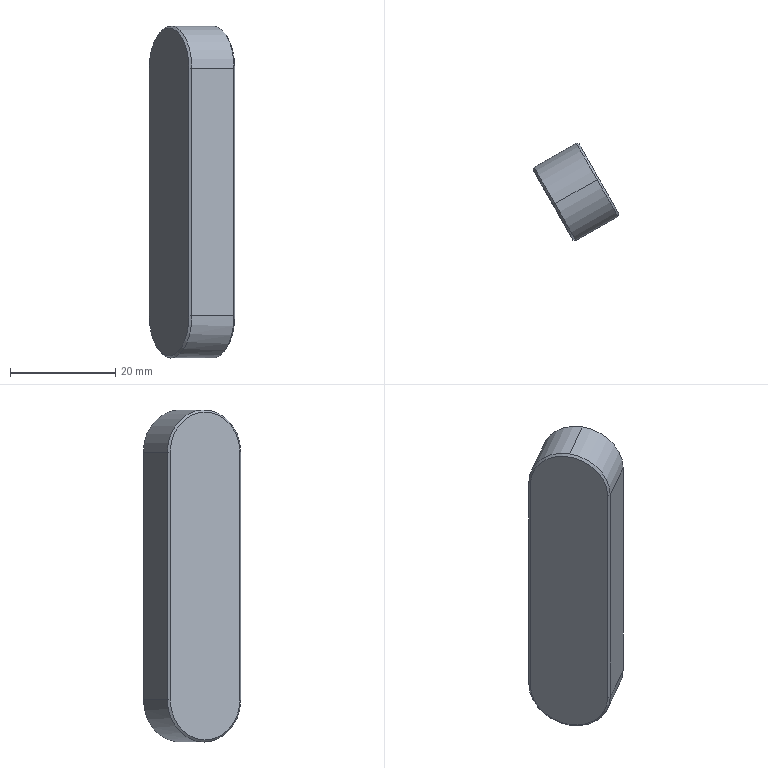Component | SolidWorks | Key16-10-63-1 | 1 solid | 17 faces | box 16.22 x 18.46 x 63 mm | volume 9508 mm3 | plane 8 | cone 6 | cylinder 3 | commonest cylinder face diameters 16 x3
build123d program:
from build123d import *

# Parameters (mm, degrees)
BOSS_EXTRUDE1_DEPTH = 10
CHAMFER1_SIZE2      = 0.4
CHAMFER1_SIZE       = 0.4


with BuildPart() as part:
    # Sketch1 → Boss-Extrude1 (new body)
    with BuildSketch(Plane(origin=(0, 0, 4), x_dir=(1, 0, 0), z_dir=(0, -1, 0))):
        with BuildLine():
            Line((-8, 43), (-8, -4))
            ThreePointArc((-8, -4), (0, -12), (8, -4))
            Line((8, -4), (8, 43))
            ThreePointArc((8, 43), (0, 51), (-8, 43))
        make_face()
    extrude(amount=-BOSS_EXTRUDE1_DEPTH)

    # Chamfer1
    chamfer1_edges = [part.edges().sort_by_distance(p)[0] for p in [
        (0, 10, -8),
        (8, 10, 23.5),
        (0, 10, 55),
        (8, 0, 23.5),
        (0, 0, -8),
        (-8, 0, 23.5),
        (0, 0, 55),
        (-8, 10, 23.5),
    ]]
    chamfer(chamfer1_edges, length=CHAMFER1_SIZE, length2=CHAMFER1_SIZE2)


solid = part.part

# Placed as in the assembly
solid = solid.moved(Location((-58.232, -16.1, 50.729), (180, 0, -119.696)))
STEP:
#1=CARTESIAN_POINT('',(-1.951,-0.4388,2.296));
#2=VERTEX_POINT('',#1);
#3=CARTESIAN_POINT('',(-1.802,-0.6987,1.997));
#4=VERTEX_POINT('',#3);
#5=CARTESIAN_POINT('',(-1.951,-0.4388,1.997));
#6=DIRECTION('',(0.8687,0.4954,0.));
#7=DIRECTION('',(-0.,-0.,1.));
#8=AXIS2_PLACEMENT_3D('',#5,#6,#7);
#9=CIRCLE('',#8,0.2992);
#10=EDGE_CURVE('',#2,#4,#9,.T.);
#11=ORIENTED_EDGE('',*,*,#10,.F.);
#12=CARTESIAN_POINT('',(-1.964,-0.4466,2.312));
#13=VERTEX_POINT('',#12);
#14=CARTESIAN_POINT('',(-1.964,-0.4466,2.312));
#15=DIRECTION('',(-0.6142,-0.3503,0.7071));
#16=VECTOR('',#15,39.37);
#17=LINE('',#14,#16);
#18=EDGE_CURVE('',#2,#13,#17,.T.);
#19=ORIENTED_EDGE('',*,*,#18,.T.);
#20=CARTESIAN_POINT('',(-1.808,-0.7202,1.997));
#21=VERTEX_POINT('',#20);
#22=CARTESIAN_POINT('',(-1.964,-0.4466,1.997));
#23=DIRECTION('',(-0.8687,-0.4954,-0.));
#24=DIRECTION('',(-0.,-0.,1.));
#25=AXIS2_PLACEMENT_3D('',#22,#23,#24);
#26=CIRCLE('',#25,0.315);
#27=EDGE_CURVE('',#21,#13,#26,.T.);
#28=ORIENTED_EDGE('',*,*,#27,.F.);
#29=CARTESIAN_POINT('',(-1.802,-0.6987,1.997));
#30=DIRECTION('',(-0.2639,-0.9645,-0.));
#31=VECTOR('',#30,39.37);
#32=LINE('',#29,#31);
#33=EDGE_CURVE('',#4,#21,#32,.T.);
#34=ORIENTED_EDGE('',*,*,#33,.F.);
#35=EDGE_LOOP('',(#11,#19,#28,#34));
#36=FACE_OUTER_BOUND('',#35,.T.);
#37=CARTESIAN_POINT('',(-1.964,-0.4466,1.997));
#38=DIRECTION('',(-0.8687,-0.4954,-0.));
#39=DIRECTION('',(-0.,-0.,1.));
#40=AXIS2_PLACEMENT_3D('',#37,#38,#39);
#41=CONICAL_SURFACE('',#40,0.315,0.7854);
#42=ADVANCED_FACE('',(#36),#41,.T.);
#43=CARTESIAN_POINT('',(-2.293,-0.6339,-0.1524));
#44=VERTEX_POINT('',#43);
#45=CARTESIAN_POINT('',(-2.144,-0.8938,0.1468));
#46=VERTEX_POINT('',#45);
#47=CARTESIAN_POINT('',(-2.293,-0.6339,0.1468));
#48=DIRECTION('',(-0.8687,-0.4954,-0.));
#49=DIRECTION('',(-0.,-0.,1.));
#50=AXIS2_PLACEMENT_3D('',#47,#48,#49);
#51=CIRCLE('',#50,0.2992);
#52=EDGE_CURVE('',#44,#46,#51,.T.);
#53=ORIENTED_EDGE('',*,*,#52,.F.);
#54=CARTESIAN_POINT('',(-2.279,-0.6261,-0.1682));
#55=VERTEX_POINT('',#54);
#56=CARTESIAN_POINT('',(-2.293,-0.6339,-0.1524));
#57=DIRECTION('',(0.6142,0.3503,-0.7071));
#58=VECTOR('',#57,39.37);
#59=LINE('',#56,#58);
#60=EDGE_CURVE('',#44,#55,#59,.T.);
#61=ORIENTED_EDGE('',*,*,#60,.T.);
#62=CARTESIAN_POINT('',(-2.123,-0.8997,0.1468));
#63=VERTEX_POINT('',#62);
#64=CARTESIAN_POINT('',(-2.279,-0.6261,0.1468));
#65=DIRECTION('',(0.8687,0.4954,0.));
#66=DIRECTION('',(-0.,-0.,1.));
#67=AXIS2_PLACEMENT_3D('',#64,#65,#66);
#68=CIRCLE('',#67,0.315);
#69=EDGE_CURVE('',#63,#55,#68,.T.);
#70=ORIENTED_EDGE('',*,*,#69,.F.);
#71=CARTESIAN_POINT('',(-2.123,-0.8997,0.1468));
#72=DIRECTION('',(-0.9645,0.2639,-0.));
#73=VECTOR('',#72,39.37);
#74=LINE('',#71,#73);
#75=EDGE_CURVE('',#63,#46,#74,.T.);
#76=ORIENTED_EDGE('',*,*,#75,.T.);
#77=EDGE_LOOP('',(#53,#61,#70,#76));
#78=FACE_OUTER_BOUND('',#77,.T.);
#79=CARTESIAN_POINT('',(-2.293,-0.6339,0.1468));
#80=DIRECTION('',(0.8687,0.4954,0.));
#81=DIRECTION('',(0.,0.,-1.));
#82=AXIS2_PLACEMENT_3D('',#79,#80,#81);
#83=CONICAL_SURFACE('',#82,0.2992,0.7854);
#84=ADVANCED_FACE('',(#78),#83,.T.);
#85=ORIENTED_EDGE('',*,*,#27,.T.);
#86=CARTESIAN_POINT('',(-2.279,-0.6261,2.312));
#87=VERTEX_POINT('',#86);
#88=CARTESIAN_POINT('',(-1.951,-0.4388,2.312));
#89=DIRECTION('',(-0.8687,-0.4954,-0.));
#90=VECTOR('',#89,39.37);
#91=LINE('',#88,#90);
#92=EDGE_CURVE('',#13,#87,#91,.T.);
#93=ORIENTED_EDGE('',*,*,#92,.T.);
#94=CARTESIAN_POINT('',(-2.123,-0.8997,1.997));
#95=VERTEX_POINT('',#94);
#96=CARTESIAN_POINT('',(-2.279,-0.6261,1.997));
#97=DIRECTION('',(0.8687,0.4954,0.));
#98=DIRECTION('',(-0.,-0.,1.));
#99=AXIS2_PLACEMENT_3D('',#96,#97,#98);
#100=CIRCLE('',#99,0.315);
#101=EDGE_CURVE('',#87,#95,#100,.T.);
#102=ORIENTED_EDGE('',*,*,#101,.T.);
#103=CARTESIAN_POINT('',(-1.795,-0.7124,1.997));
#104=DIRECTION('',(-0.8687,-0.4954,-0.));
#105=VECTOR('',#104,39.37);
#106=LINE('',#103,#105);
#107=EDGE_CURVE('',#21,#95,#106,.T.);
#108=ORIENTED_EDGE('',*,*,#107,.F.);
#109=EDGE_LOOP('',(#85,#93,#102,#108));
#110=FACE_OUTER_BOUND('',#109,.T.);
#111=CARTESIAN_POINT('',(-1.951,-0.4388,1.997));
#112=DIRECTION('',(-0.8687,-0.4954,-0.));
#113=DIRECTION('',(-0.,-0.,1.));
#114=AXIS2_PLACEMENT_3D('',#111,#112,#113);
#115=CYLINDRICAL_SURFACE('',#114,0.315);
#116=ADVANCED_FACE('',(#110),#115,.T.);
#117=CARTESIAN_POINT('',(-1.808,-0.7202,0.1468));
#118=VERTEX_POINT('',#117);
#119=CARTESIAN_POINT('',(-1.795,-0.7124,0.1468));
#120=DIRECTION('',(-0.8687,-0.4954,-0.));
#121=VECTOR('',#120,39.37);
#122=LINE('',#119,#121);
#123=EDGE_CURVE('',#118,#63,#122,.T.);
#124=ORIENTED_EDGE('',*,*,#123,.T.);
#125=ORIENTED_EDGE('',*,*,#69,.T.);
#126=CARTESIAN_POINT('',(-2.435,-0.3525,0.1468));
#127=VERTEX_POINT('',#126);
#128=CARTESIAN_POINT('',(-2.279,-0.6261,0.1468));
#129=DIRECTION('',(0.8687,0.4954,0.));
#130=DIRECTION('',(-0.,-0.,1.));
#131=AXIS2_PLACEMENT_3D('',#128,#129,#130);
#132=CIRCLE('',#131,0.315);
#133=EDGE_CURVE('',#55,#127,#132,.T.);
#134=ORIENTED_EDGE('',*,*,#133,.T.);
#135=CARTESIAN_POINT('',(-2.12,-0.173,0.1468));
#136=VERTEX_POINT('',#135);
#137=CARTESIAN_POINT('',(-2.107,-0.1652,0.1468));
#138=DIRECTION('',(-0.8687,-0.4954,-0.));
#139=VECTOR('',#138,39.37);
#140=LINE('',#137,#139);
#141=EDGE_CURVE('',#136,#127,#140,.T.);
#142=ORIENTED_EDGE('',*,*,#141,.F.);
#143=CARTESIAN_POINT('',(-1.964,-0.4466,0.1468));
#144=DIRECTION('',(-0.8687,-0.4954,-0.));
#145=DIRECTION('',(-0.,-0.,1.));
#146=AXIS2_PLACEMENT_3D('',#143,#144,#145);
#147=CIRCLE('',#146,0.315);
#148=EDGE_CURVE('',#136,#118,#147,.T.);
#149=ORIENTED_EDGE('',*,*,#148,.T.);
#150=EDGE_LOOP('',(#124,#125,#134,#142,#149));
#151=FACE_OUTER_BOUND('',#150,.T.);
#152=CARTESIAN_POINT('',(-1.951,-0.4388,0.1468));
#153=DIRECTION('',(-0.8687,-0.4954,-0.));
#154=DIRECTION('',(-0.,-0.,1.));
#155=AXIS2_PLACEMENT_3D('',#152,#153,#154);
#156=CYLINDRICAL_SURFACE('',#155,0.315);
#157=ADVANCED_FACE('',(#151),#156,.T.);
#158=ORIENTED_EDGE('',*,*,#141,.T.);
#159=CARTESIAN_POINT('',(-2.435,-0.3525,1.997));
#160=VERTEX_POINT('',#159);
#161=CARTESIAN_POINT('',(-2.435,-0.3525,1.997));
#162=DIRECTION('',(-0.,-0.,1.));
#163=VECTOR('',#162,39.37);
#164=LINE('',#161,#163);
#165=EDGE_CURVE('',#127,#160,#164,.T.);
#166=ORIENTED_EDGE('',*,*,#165,.T.);
#167=CARTESIAN_POINT('',(-2.12,-0.173,1.997));
#168=VERTEX_POINT('',#167);
#169=CARTESIAN_POINT('',(-2.107,-0.1652,1.997));
#170=DIRECTION('',(-0.8687,-0.4954,-0.));
#171=VECTOR('',#170,39.37);
#172=LINE('',#169,#171);
#173=EDGE_CURVE('',#168,#160,#172,.T.);
#174=ORIENTED_EDGE('',*,*,#173,.F.);
#175=CARTESIAN_POINT('',(-2.12,-0.173,0.1468));
#176=DIRECTION('',(0.,0.,-1.));
#177=VECTOR('',#176,39.37);
#178=LINE('',#175,#177);
#179=EDGE_CURVE('',#168,#136,#178,.T.);
#180=ORIENTED_EDGE('',*,*,#179,.T.);
#181=EDGE_LOOP('',(#158,#166,#174,#180));
#182=FACE_OUTER_BOUND('',#181,.T.);
#183=CARTESIAN_POINT('',(-2.107,-0.1652,1.997));
#184=DIRECTION('',(-0.4954,0.8687,-0.));
#185=DIRECTION('',(-0.,-0.,1.));
#186=AXIS2_PLACEMENT_3D('',#183,#184,#185);
#187=PLANE('',#186);
#188=ADVANCED_FACE('',(#182),#187,.T.);
#189=ORIENTED_EDGE('',*,*,#92,.F.);
#190=CARTESIAN_POINT('',(-1.964,-0.4466,1.997));
#191=DIRECTION('',(-0.8687,-0.4954,-0.));
#192=DIRECTION('',(-0.,-0.,1.));
#193=AXIS2_PLACEMENT_3D('',#190,#191,#192);
#194=CIRCLE('',#193,0.315);
#195=EDGE_CURVE('',#13,#168,#194,.T.);
#196=ORIENTED_EDGE('',*,*,#195,.T.);
#197=ORIENTED_EDGE('',*,*,#173,.T.);
#198=CARTESIAN_POINT('',(-2.279,-0.6261,1.997));
#199=DIRECTION('',(0.8687,0.4954,0.));
#200=DIRECTION('',(-0.,0.,1.));
#201=AXIS2_PLACEMENT_3D('',#198,#199,#200);
#202=CIRCLE('',#201,0.315);
#203=EDGE_CURVE('',#160,#87,#202,.T.);
#204=ORIENTED_EDGE('',*,*,#203,.T.);
#205=EDGE_LOOP('',(#189,#196,#197,#204));
#206=FACE_OUTER_BOUND('',#205,.T.);
#207=CARTESIAN_POINT('',(-1.951,-0.4388,1.997));
#208=DIRECTION('',(-0.8687,-0.4954,-0.));
#209=DIRECTION('',(-0.,-0.,1.));
#210=AXIS2_PLACEMENT_3D('',#207,#208,#209);
#211=CYLINDRICAL_SURFACE('',#210,0.315);
#212=ADVANCED_FACE('',(#206),#211,.T.);
#213=ORIENTED_EDGE('',*,*,#107,.T.);
#214=CARTESIAN_POINT('',(-2.123,-0.8997,0.1468));
#215=DIRECTION('',(0.,0.,-1.));
#216=VECTOR('',#215,39.37);
#217=LINE('',#214,#216);
#218=EDGE_CURVE('',#95,#63,#217,.T.);
#219=ORIENTED_EDGE('',*,*,#218,.T.);
#220=ORIENTED_EDGE('',*,*,#123,.F.);
#221=CARTESIAN_POINT('',(-1.808,-0.7202,1.997));
#222=DIRECTION('',(-0.,-0.,1.));
#223=VECTOR('',#222,39.37);
#224=LINE('',#221,#223);
#225=EDGE_CURVE('',#118,#21,#224,.T.);
#226=ORIENTED_EDGE('',*,*,#225,.T.);
#227=EDGE_LOOP('',(#213,#219,#220,#226));
#228=FACE_OUTER_BOUND('',#227,.T.);
#229=CARTESIAN_POINT('',(-1.795,-0.7124,0.1468));
#230=DIRECTION('',(0.4954,-0.8687,0.));
#231=DIRECTION('',(0.,0.,-1.));
#232=AXIS2_PLACEMENT_3D('',#229,#230,#231);
#233=PLANE('',#232);
#234=ADVANCED_FACE('',(#228),#233,.T.);
#235=CARTESIAN_POINT('',(-2.099,-0.1789,1.997));
#236=VERTEX_POINT('',#235);
#237=CARTESIAN_POINT('',(-1.951,-0.4388,1.997));
#238=DIRECTION('',(0.8687,0.4954,0.));
#239=DIRECTION('',(-0.,-0.,1.));
#240=AXIS2_PLACEMENT_3D('',#237,#238,#239);
#241=CIRCLE('',#240,0.2992);
#242=EDGE_CURVE('',#236,#2,#241,.T.);
#243=ORIENTED_EDGE('',*,*,#242,.T.);
#244=ORIENTED_EDGE('',*,*,#10,.T.);
#245=CARTESIAN_POINT('',(-1.802,-0.6987,0.1468));
#246=VERTEX_POINT('',#245);
#247=CARTESIAN_POINT('',(-1.802,-0.6987,0.1468));
#248=DIRECTION('',(0.,0.,-1.));
#249=VECTOR('',#248,39.37);
#250=LINE('',#247,#249);
#251=EDGE_CURVE('',#4,#246,#250,.T.);
#252=ORIENTED_EDGE('',*,*,#251,.T.);
#253=CARTESIAN_POINT('',(-2.099,-0.1789,0.1468));
#254=VERTEX_POINT('',#253);
#255=CARTESIAN_POINT('',(-1.951,-0.4388,0.1468));
#256=DIRECTION('',(0.8687,0.4954,0.));
#257=DIRECTION('',(-0.,0.,1.));
#258=AXIS2_PLACEMENT_3D('',#255,#256,#257);
#259=CIRCLE('',#258,0.2992);
#260=EDGE_CURVE('',#246,#254,#259,.T.);
#261=ORIENTED_EDGE('',*,*,#260,.T.);
#262=CARTESIAN_POINT('',(-2.099,-0.1789,1.997));
#263=DIRECTION('',(-0.,-0.,1.));
#264=VECTOR('',#263,39.37);
#265=LINE('',#262,#264);
#266=EDGE_CURVE('',#254,#236,#265,.T.);
#267=ORIENTED_EDGE('',*,*,#266,.T.);
#268=EDGE_LOOP('',(#243,#244,#252,#261,#267));
#269=FACE_OUTER_BOUND('',#268,.T.);
#270=CARTESIAN_POINT('',(-1.951,-0.4388,0.1468));
#271=DIRECTION('',(-0.8687,-0.4954,-0.));
#272=DIRECTION('',(-0.,-0.,1.));
#273=AXIS2_PLACEMENT_3D('',#270,#271,#272);
#274=PLANE('',#273);
#275=ADVANCED_FACE('',(#269),#274,.F.);
#276=CARTESIAN_POINT('',(-2.144,-0.8938,1.997));
#277=VERTEX_POINT('',#276);
#278=CARTESIAN_POINT('',(-2.441,-0.374,1.997));
#279=VERTEX_POINT('',#278);
#280=CARTESIAN_POINT('',(-2.293,-0.6339,1.997));
#281=DIRECTION('',(-0.8687,-0.4954,-0.));
#282=DIRECTION('',(-0.,-0.,1.));
#283=AXIS2_PLACEMENT_3D('',#280,#281,#282);
#284=CIRCLE('',#283,0.2992);
#285=EDGE_CURVE('',#277,#279,#284,.T.);
#286=ORIENTED_EDGE('',*,*,#285,.T.);
#287=CARTESIAN_POINT('',(-2.441,-0.374,0.1468));
#288=VERTEX_POINT('',#287);
#289=CARTESIAN_POINT('',(-2.441,-0.374,0.1468));
#290=DIRECTION('',(0.,0.,-1.));
#291=VECTOR('',#290,39.37);
#292=LINE('',#289,#291);
#293=EDGE_CURVE('',#279,#288,#292,.T.);
#294=ORIENTED_EDGE('',*,*,#293,.T.);
#295=CARTESIAN_POINT('',(-2.293,-0.6339,0.1468));
#296=DIRECTION('',(-0.8687,-0.4954,-0.));
#297=DIRECTION('',(-0.,-0.,1.));
#298=AXIS2_PLACEMENT_3D('',#295,#296,#297);
#299=CIRCLE('',#298,0.2992);
#300=EDGE_CURVE('',#288,#44,#299,.T.);
#301=ORIENTED_EDGE('',*,*,#300,.T.);
#302=ORIENTED_EDGE('',*,*,#52,.T.);
#303=CARTESIAN_POINT('',(-2.144,-0.8938,0.1468));
#304=DIRECTION('',(-0.,-0.,1.));
#305=VECTOR('',#304,39.37);
#306=LINE('',#303,#305);
#307=EDGE_CURVE('',#46,#277,#306,.T.);
#308=ORIENTED_EDGE('',*,*,#307,.T.);
#309=EDGE_LOOP('',(#286,#294,#301,#302,#308));
#310=FACE_OUTER_BOUND('',#309,.T.);
#311=CARTESIAN_POINT('',(-2.293,-0.6339,0.1468));
#312=DIRECTION('',(-0.8687,-0.4954,-0.));
#313=DIRECTION('',(-0.,-0.,1.));
#314=AXIS2_PLACEMENT_3D('',#311,#312,#313);
#315=PLANE('',#314);
#316=ADVANCED_FACE('',(#310),#315,.T.);
#317=ORIENTED_EDGE('',*,*,#75,.F.);
#318=ORIENTED_EDGE('',*,*,#218,.F.);
#319=CARTESIAN_POINT('',(-2.144,-0.8938,1.997));
#320=DIRECTION('',(0.9645,-0.2639,0.));
#321=VECTOR('',#320,39.37);
#322=LINE('',#319,#321);
#323=EDGE_CURVE('',#277,#95,#322,.T.);
#324=ORIENTED_EDGE('',*,*,#323,.F.);
#325=ORIENTED_EDGE('',*,*,#307,.F.);
#326=EDGE_LOOP('',(#317,#318,#324,#325));
#327=FACE_OUTER_BOUND('',#326,.T.);
#328=CARTESIAN_POINT('',(-2.144,-0.8938,0.1468));
#329=DIRECTION('',(0.2639,0.9645,0.));
#330=DIRECTION('',(-0.,-0.,1.));
#331=AXIS2_PLACEMENT_3D('',#328,#329,#330);
#332=PLANE('',#331);
#333=ADVANCED_FACE('',(#327),#332,.F.);
#334=ORIENTED_EDGE('',*,*,#323,.T.);
#335=ORIENTED_EDGE('',*,*,#101,.F.);
#336=ORIENTED_EDGE('',*,*,#203,.F.);
#337=CARTESIAN_POINT('',(-2.441,-0.374,1.997));
#338=DIRECTION('',(0.2639,0.9645,0.));
#339=VECTOR('',#338,39.37);
#340=LINE('',#337,#339);
#341=EDGE_CURVE('',#279,#160,#340,.T.);
#342=ORIENTED_EDGE('',*,*,#341,.F.);
#343=ORIENTED_EDGE('',*,*,#285,.F.);
#344=EDGE_LOOP('',(#334,#335,#336,#342,#343));
#345=FACE_OUTER_BOUND('',#344,.T.);
#346=CARTESIAN_POINT('',(-2.293,-0.6339,1.997));
#347=DIRECTION('',(0.8687,0.4954,0.));
#348=DIRECTION('',(0.,0.,-1.));
#349=AXIS2_PLACEMENT_3D('',#346,#347,#348);
#350=CONICAL_SURFACE('',#349,0.2992,0.7854);
#351=ADVANCED_FACE('',(#345),#350,.T.);
#352=ORIENTED_EDGE('',*,*,#60,.F.);
#353=ORIENTED_EDGE('',*,*,#300,.F.);
#354=CARTESIAN_POINT('',(-2.435,-0.3525,0.1468));
#355=DIRECTION('',(-0.2639,-0.9645,-0.));
#356=VECTOR('',#355,39.37);
#357=LINE('',#354,#356);
#358=EDGE_CURVE('',#127,#288,#357,.T.);
#359=ORIENTED_EDGE('',*,*,#358,.F.);
#360=ORIENTED_EDGE('',*,*,#133,.F.);
#361=EDGE_LOOP('',(#352,#353,#359,#360));
#362=FACE_OUTER_BOUND('',#361,.T.);
#363=CARTESIAN_POINT('',(-2.293,-0.6339,0.1468));
#364=DIRECTION('',(0.8687,0.4954,0.));
#365=DIRECTION('',(0.,0.,-1.));
#366=AXIS2_PLACEMENT_3D('',#363,#364,#365);
#367=CONICAL_SURFACE('',#366,0.2992,0.7854);
#368=ADVANCED_FACE('',(#362),#367,.T.);
#369=ORIENTED_EDGE('',*,*,#341,.T.);
#370=ORIENTED_EDGE('',*,*,#165,.F.);
#371=ORIENTED_EDGE('',*,*,#358,.T.);
#372=ORIENTED_EDGE('',*,*,#293,.F.);
#373=EDGE_LOOP('',(#369,#370,#371,#372));
#374=FACE_OUTER_BOUND('',#373,.T.);
#375=CARTESIAN_POINT('',(-2.441,-0.374,0.1468));
#376=DIRECTION('',(0.9645,-0.2639,0.));
#377=DIRECTION('',(0.,0.,-1.));
#378=AXIS2_PLACEMENT_3D('',#375,#376,#377);
#379=PLANE('',#378);
#380=ADVANCED_FACE('',(#374),#379,.F.);
#381=CARTESIAN_POINT('',(-2.099,-0.1789,1.997));
#382=DIRECTION('',(-0.9645,0.2639,-0.));
#383=VECTOR('',#382,39.37);
#384=LINE('',#381,#383);
#385=EDGE_CURVE('',#236,#168,#384,.T.);
#386=ORIENTED_EDGE('',*,*,#385,.F.);
#387=ORIENTED_EDGE('',*,*,#266,.F.);
#388=CARTESIAN_POINT('',(-2.12,-0.173,0.1468));
#389=DIRECTION('',(0.9645,-0.2639,0.));
#390=VECTOR('',#389,39.37);
#391=LINE('',#388,#390);
#392=EDGE_CURVE('',#136,#254,#391,.T.);
#393=ORIENTED_EDGE('',*,*,#392,.F.);
#394=ORIENTED_EDGE('',*,*,#179,.F.);
#395=EDGE_LOOP('',(#386,#387,#393,#394));
#396=FACE_OUTER_BOUND('',#395,.T.);
#397=CARTESIAN_POINT('',(-2.12,-0.173,1.997));
#398=DIRECTION('',(0.2639,0.9645,0.));
#399=DIRECTION('',(-0.,-0.,1.));
#400=AXIS2_PLACEMENT_3D('',#397,#398,#399);
#401=PLANE('',#400);
#402=ADVANCED_FACE('',(#396),#401,.T.);
#403=ORIENTED_EDGE('',*,*,#392,.T.);
#404=ORIENTED_EDGE('',*,*,#260,.F.);
#405=CARTESIAN_POINT('',(-1.808,-0.7202,0.1468));
#406=DIRECTION('',(0.2639,0.9645,0.));
#407=VECTOR('',#406,39.37);
#408=LINE('',#405,#407);
#409=EDGE_CURVE('',#118,#246,#408,.T.);
#410=ORIENTED_EDGE('',*,*,#409,.F.);
#411=ORIENTED_EDGE('',*,*,#148,.F.);
#412=EDGE_LOOP('',(#403,#404,#410,#411));
#413=FACE_OUTER_BOUND('',#412,.T.);
#414=CARTESIAN_POINT('',(-1.964,-0.4466,0.1468));
#415=DIRECTION('',(-0.8687,-0.4954,-0.));
#416=DIRECTION('',(-0.,-0.,1.));
#417=AXIS2_PLACEMENT_3D('',#414,#415,#416);
#418=CONICAL_SURFACE('',#417,0.315,0.7854);
#419=ADVANCED_FACE('',(#413),#418,.T.);
#420=ORIENTED_EDGE('',*,*,#18,.F.);
#421=ORIENTED_EDGE('',*,*,#242,.F.);
#422=ORIENTED_EDGE('',*,*,#385,.T.);
#423=ORIENTED_EDGE('',*,*,#195,.F.);
#424=EDGE_LOOP('',(#420,#421,#422,#423));
#425=FACE_OUTER_BOUND('',#424,.T.);
#426=CARTESIAN_POINT('',(-1.964,-0.4466,1.997));
#427=DIRECTION('',(-0.8687,-0.4954,-0.));
#428=DIRECTION('',(-0.,-0.,1.));
#429=AXIS2_PLACEMENT_3D('',#426,#427,#428);
#430=CONICAL_SURFACE('',#429,0.315,0.7854);
#431=ADVANCED_FACE('',(#425),#430,.T.);
#432=ORIENTED_EDGE('',*,*,#409,.T.);
#433=ORIENTED_EDGE('',*,*,#251,.F.);
#434=ORIENTED_EDGE('',*,*,#33,.T.);
#435=ORIENTED_EDGE('',*,*,#225,.F.);
#436=EDGE_LOOP('',(#432,#433,#434,#435));
#437=FACE_OUTER_BOUND('',#436,.T.);
#438=CARTESIAN_POINT('',(-1.808,-0.7202,0.1468));
#439=DIRECTION('',(0.9645,-0.2639,0.));
#440=DIRECTION('',(0.,0.,-1.));
#441=AXIS2_PLACEMENT_3D('',#438,#439,#440);
#442=PLANE('',#441);
#443=ADVANCED_FACE('',(#437),#442,.T.);
#444=CLOSED_SHELL('',(#42,#84,#116,#157,#188,#212,#234,#275,#316,#333,#351,#368,#380,#402,#419,#431,#443));
#445=MANIFOLD_SOLID_BREP('',#444);
#446=CARTESIAN_POINT('',(0.,0.,0.));
#447=DIRECTION('',(0.,0.,1.));
#448=DIRECTION('',(1.,0.,0.));
#449=AXIS2_PLACEMENT_3D('',#446,#447,#448);
#450=(LENGTH_UNIT()NAMED_UNIT(*)SI_UNIT($,.METRE.));
#451=LENGTH_MEASURE_WITH_UNIT(LENGTH_MEASURE(0.0254),#450);
#452=DIMENSIONAL_EXPONENTS(1.,0.,0.,0.,0.,0.,0.);
#453=(CONVERSION_BASED_UNIT('',#451)LENGTH_UNIT()NAMED_UNIT(#452));
#454=UNCERTAINTY_MEASURE_WITH_UNIT(LENGTH_MEASURE(0.00001),#453,'','');
#455=(NAMED_UNIT(*)PLANE_ANGLE_UNIT()SI_UNIT($,.RADIAN.));
#456=(NAMED_UNIT(*)SI_UNIT($,.STERADIAN.)SOLID_ANGLE_UNIT());
#457=(GEOMETRIC_REPRESENTATION_CONTEXT(3)GLOBAL_UNCERTAINTY_ASSIGNED_CONTEXT((#454))GLOBAL_UNIT_ASSIGNED_CONTEXT((#453,#455,#456))REPRESENTATION_CONTEXT('',''));
#458=ADVANCED_BREP_SHAPE_REPRESENTATION('',(#445,#449),#457);
#459=COLOUR_RGB('',0.7922,0.8196,0.9333);
#460=FILL_AREA_STYLE_COLOUR('',#459);
#461=FILL_AREA_STYLE('',(#460));
#462=SURFACE_STYLE_FILL_AREA(#461);
#463=SURFACE_SIDE_STYLE('',(#462));
#464=SURFACE_STYLE_USAGE(.BOTH.,#463);
#465=PRESENTATION_STYLE_ASSIGNMENT((#464));
#466=STYLED_ITEM('',(#465),#445);
#467=(LENGTH_UNIT()NAMED_UNIT(*)SI_UNIT($,.METRE.));
#468=LENGTH_MEASURE_WITH_UNIT(LENGTH_MEASURE(0.0254),#467);
#469=DIMENSIONAL_EXPONENTS(1.,0.,0.,0.,0.,0.,0.);
#470=(CONVERSION_BASED_UNIT('',#468)LENGTH_UNIT()NAMED_UNIT(#469));
#471=UNCERTAINTY_MEASURE_WITH_UNIT(LENGTH_MEASURE(0.00001),#470,'','');
#472=(NAMED_UNIT(*)PLANE_ANGLE_UNIT()SI_UNIT($,.RADIAN.));
#473=(NAMED_UNIT(*)SI_UNIT($,.STERADIAN.)SOLID_ANGLE_UNIT());
#474=(GEOMETRIC_REPRESENTATION_CONTEXT(3)GLOBAL_UNCERTAINTY_ASSIGNED_CONTEXT((#471))GLOBAL_UNIT_ASSIGNED_CONTEXT((#470,#472,#473))REPRESENTATION_CONTEXT('',''));
#475=MECHANICAL_DESIGN_GEOMETRIC_PRESENTATION_REPRESENTATION('',(#466),#474);
#476=PRESENTATION_LAYER_ASSIGNMENT('','',(#466));